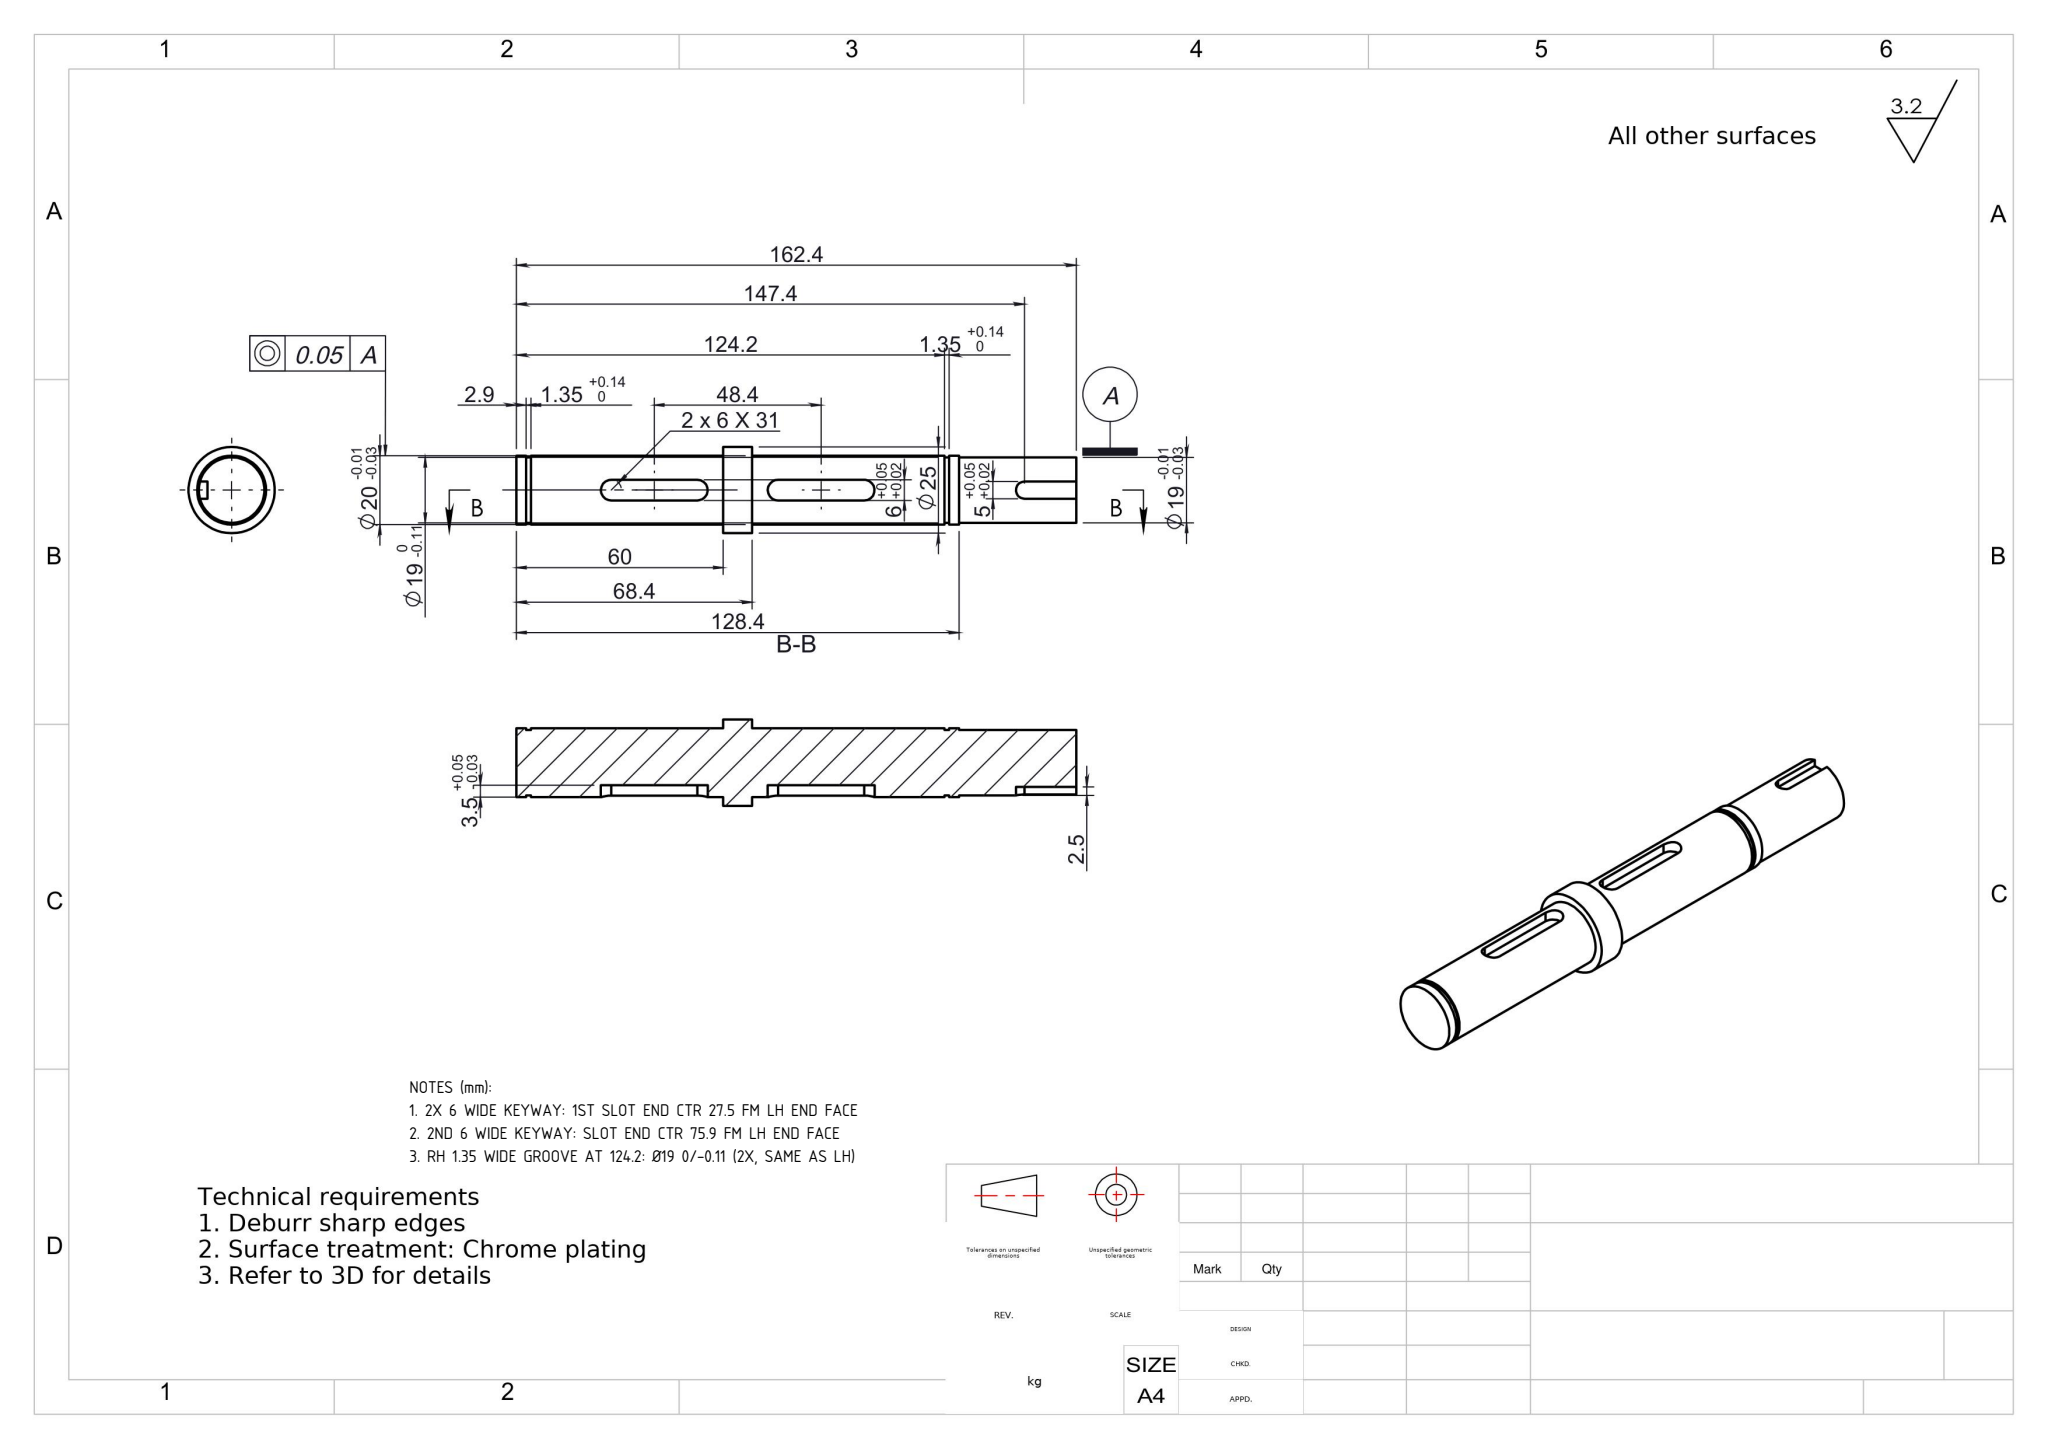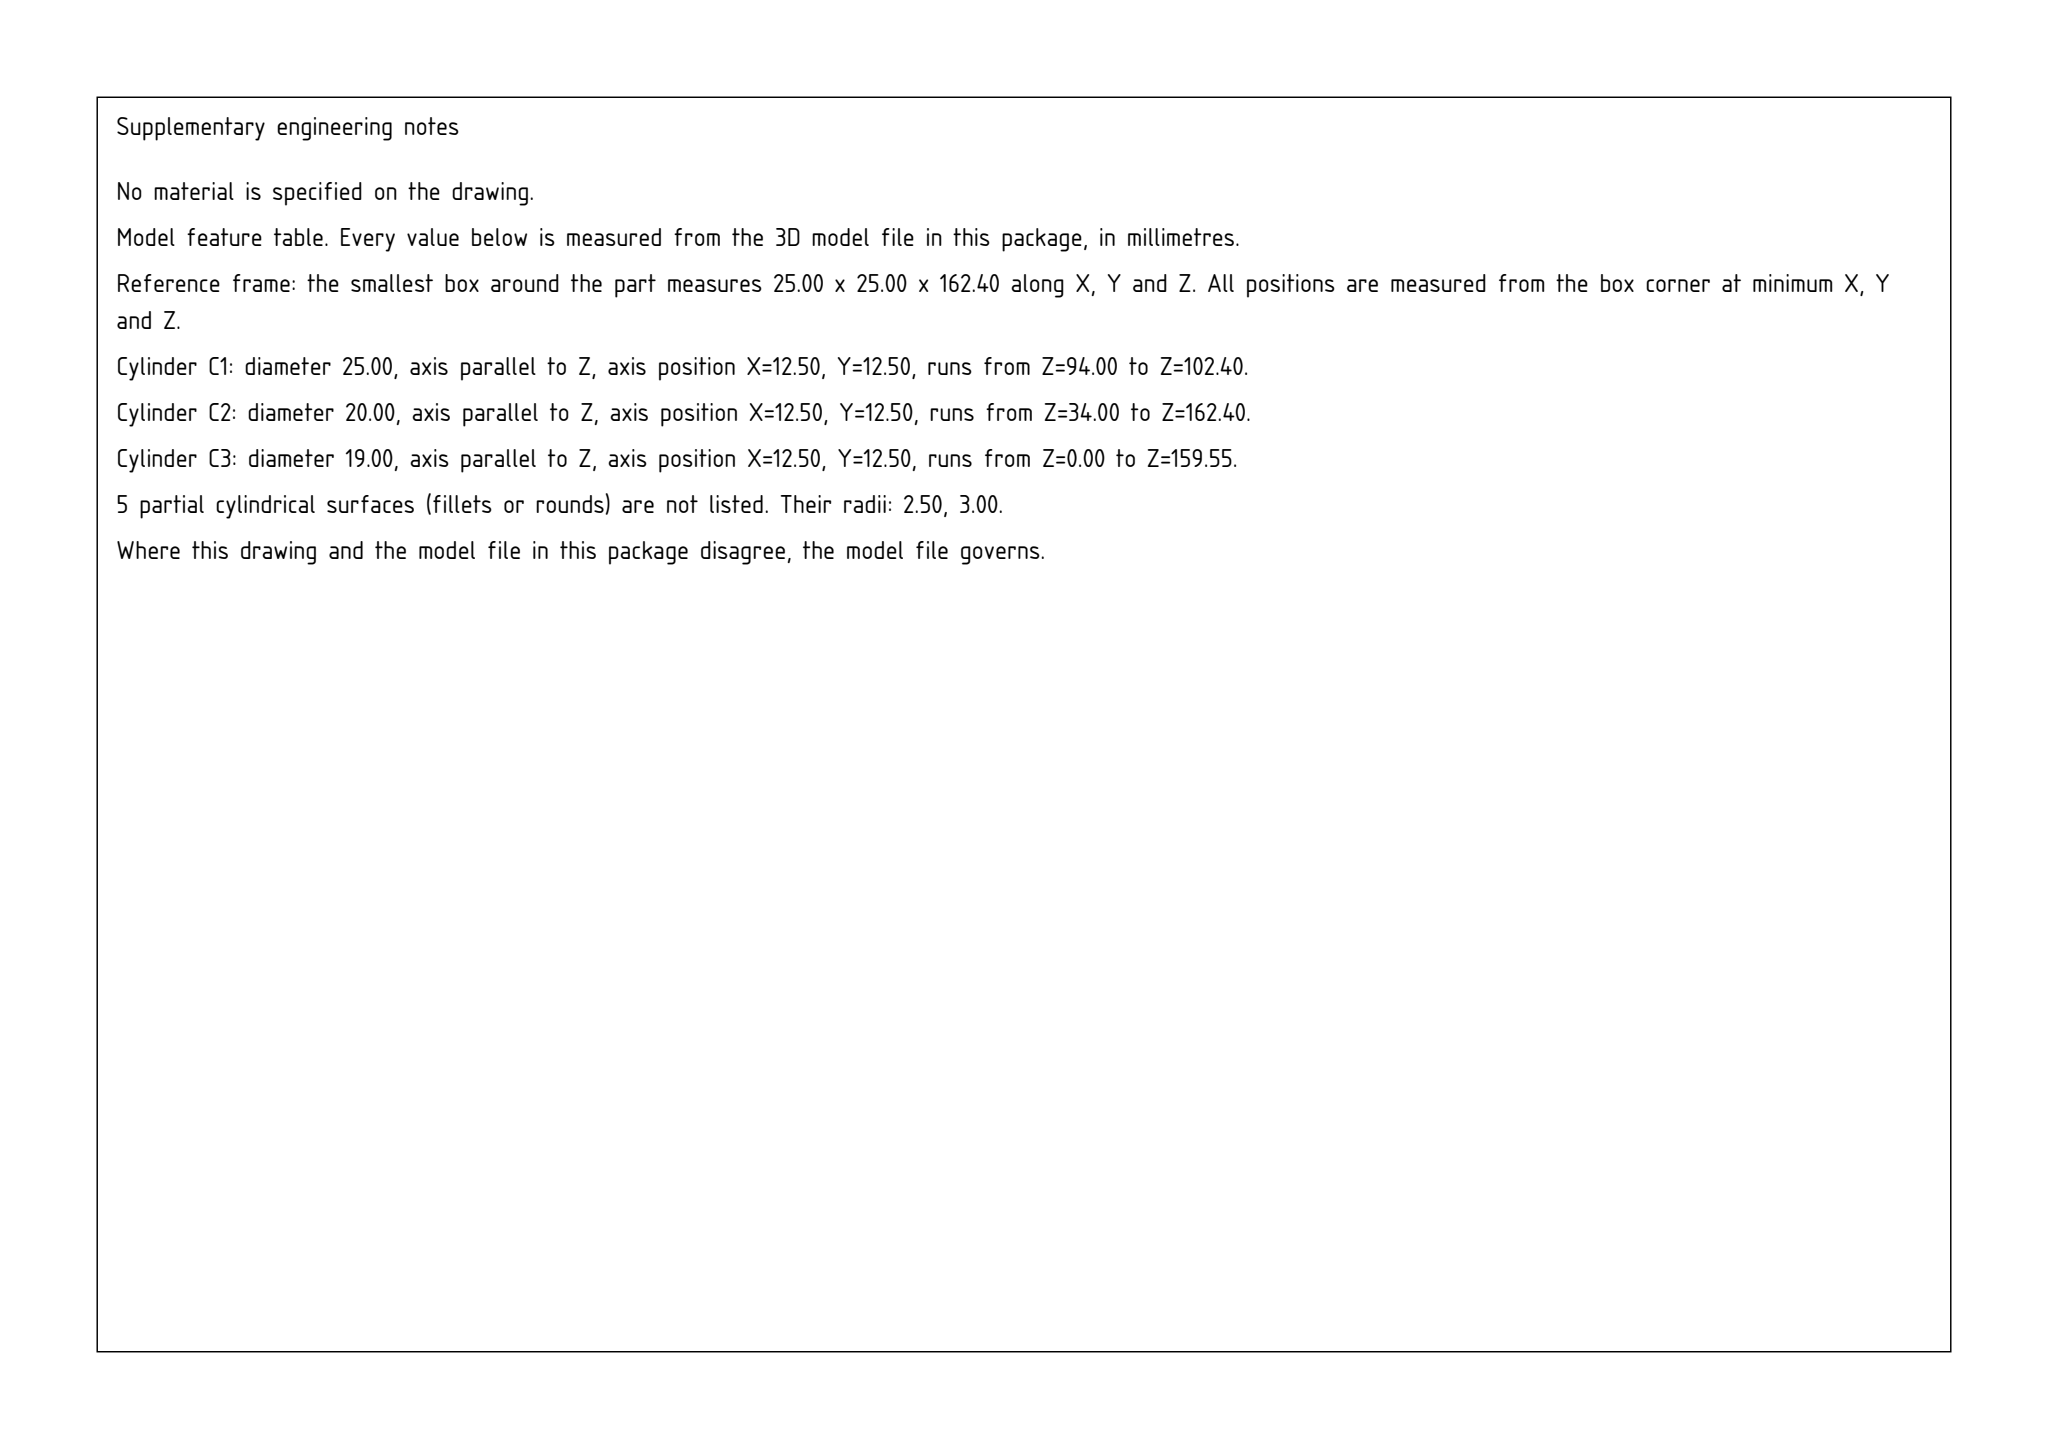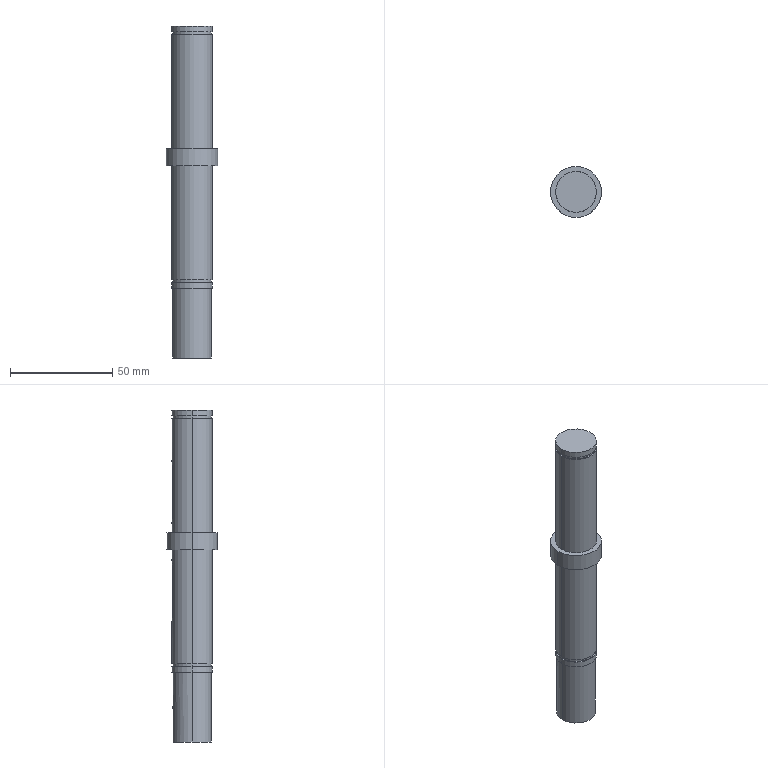Part | SolidWorks | mm | 1 solid | 42 faces | box 25 x 25 x 162.4 mm | volume 49981 mm3 | cylinder 24 | plane 18 | commonest cylinder face diameters 20 x8 6 x6 19 x6 5 x2 25 x2
Drawing notes:
2X 6 WIDE KEYWAY: 1ST SLOT END CTR 27.5 FM LH END FACE | from the solid: Ø6 end-mill cyls at z=134.9 & 109.9; LH end face z=162.4 -> 162.4-134.9=27.5 (slot ends 24.5 to 55.5, 31 lg)
2ND 6 WIDE KEYWAY: SLOT END CTR 75.9 FM LH END FACE | from the solid: Ø6 cyls at z=86.5 & 61.5; 162.4-86.5=75.9, 48.4 from 1st slot, 31 lg
RH 1.35 WIDE GROOVE AT 124.2: Ø19 0/-0.11 (2X, SAME AS LH) | from the solid: Cyl dia 19 z-axis len 1.35 spanning z=36.85-38.2 (=162.4-124.2 from LH end face z=162.4); identical to LH groove z=158.2-159.55
build123d program:
from build123d import *

# Parameters (mm, degrees)
SKETCH1_R           = 12.5
BOSS_EXTRUDE1_DEPTH = 4.2
SKETCH2_R           = 10
BOSS_EXTRUDE2_DEPTH = 60
CUT_EXTRUDE1_START  = 55.8
SKETCH3_OUTSIDE_W   = 42.4
SKETCH3_OUTSIDE_H   = 42.4
SKETCH3_OUTSIDE_R   = 9.5
CUT_EXTRUDE1_DEPTH  = 1.35
SKETCH4_R           = 9.5
BOSS_EXTRUDE3_DEPTH = 34
CUT_EXTRUDE2_DEPTH  = 2.5
CUT_EXTRUDE3_START  = 10
CUT_EXTRUDE3_DEPTH  = 3.5


with BuildPart() as part:
    # Sketch1 → Boss-Extrude1 (new, symmetric)
    with BuildSketch(Plane.XY):
        Circle(SKETCH1_R)
    extrude(amount=BOSS_EXTRUDE1_DEPTH, both=True)

    # Sketch2 → Boss-Extrude2 (add)
    with BuildSketch(Plane.XY.offset(4.2)):
        Circle(SKETCH2_R)
    boss_extrude2 = extrude(amount=BOSS_EXTRUDE2_DEPTH)

    # Sketch3 outside → Cut-Extrude1 (cut)
    with BuildSketch(Plane.XY.offset(4.2).offset(CUT_EXTRUDE1_START)):
        Rectangle(SKETCH3_OUTSIDE_W, SKETCH3_OUTSIDE_H)
        with Locations(Location((0, 0, 0), (0, 0, 180))):
            Circle(SKETCH3_OUTSIDE_R, mode=Mode.SUBTRACT)
    cut_extrude1 = extrude(amount=CUT_EXTRUDE1_DEPTH, mode=Mode.SUBTRACT)

    # Mirror1: Boss-Extrude2, Cut-Extrude1 across plane
    add(boss_extrude2.mirror(Plane.XY))
    add(cut_extrude1.mirror(Plane.XY), mode=Mode.SUBTRACT)

    # Sketch4 → Boss-Extrude3 (add)
    with BuildSketch(Plane.XY.offset(-64.2)):
        with Locations(Location((0, 0, 0), (0, 0, 180))):
            Circle(SKETCH4_R)
    extrude(amount=-BOSS_EXTRUDE3_DEPTH)

    # Sketch6 → Cut-Extrude2 (cut)
    with BuildSketch(Plane(origin=(0, 9.5, 0), x_dir=(1, 0, 0), z_dir=(0, 1, 0))):
        with BuildLine():
            Line((2.5, 98.2), (2.5, 83.2))
            ThreePointArc((2.5, 83.2), (0, 80.7), (-2.5, 83.2))
            Line((-2.5, 83.2), (-2.5, 98.2))
            ThreePointArc((-2.5, 98.2), (0, 100.7), (2.5, 98.2))
        make_face()
    extrude(amount=-CUT_EXTRUDE2_DEPTH, mode=Mode.SUBTRACT)

    # Sketch7 → Cut-Extrude3 (cut)
    with BuildSketch(Plane(origin=(0, 0, 0), x_dir=(1, 0, 0), z_dir=(0, 1, 0)).offset(CUT_EXTRUDE3_START)):
        with BuildLine():
            Line((-3, -36.7), (-3, -11.7))
            ThreePointArc((-3, -11.7), (0, -8.7), (3, -11.7))
            Line((3, -11.7), (3, -36.7))
            ThreePointArc((3, -36.7), (0, -39.7), (-3, -36.7))
        make_face()
        with BuildLine():
            Line((-3, 36.7), (-3, 11.7))
            ThreePointArc((-3, 11.7), (0, 8.7), (3, 11.7))
            Line((3, 11.7), (3, 36.7))
            ThreePointArc((3, 36.7), (0, 39.7), (-3, 36.7))
        make_face()
    extrude(amount=-CUT_EXTRUDE3_DEPTH, mode=Mode.SUBTRACT)


solid = part.part